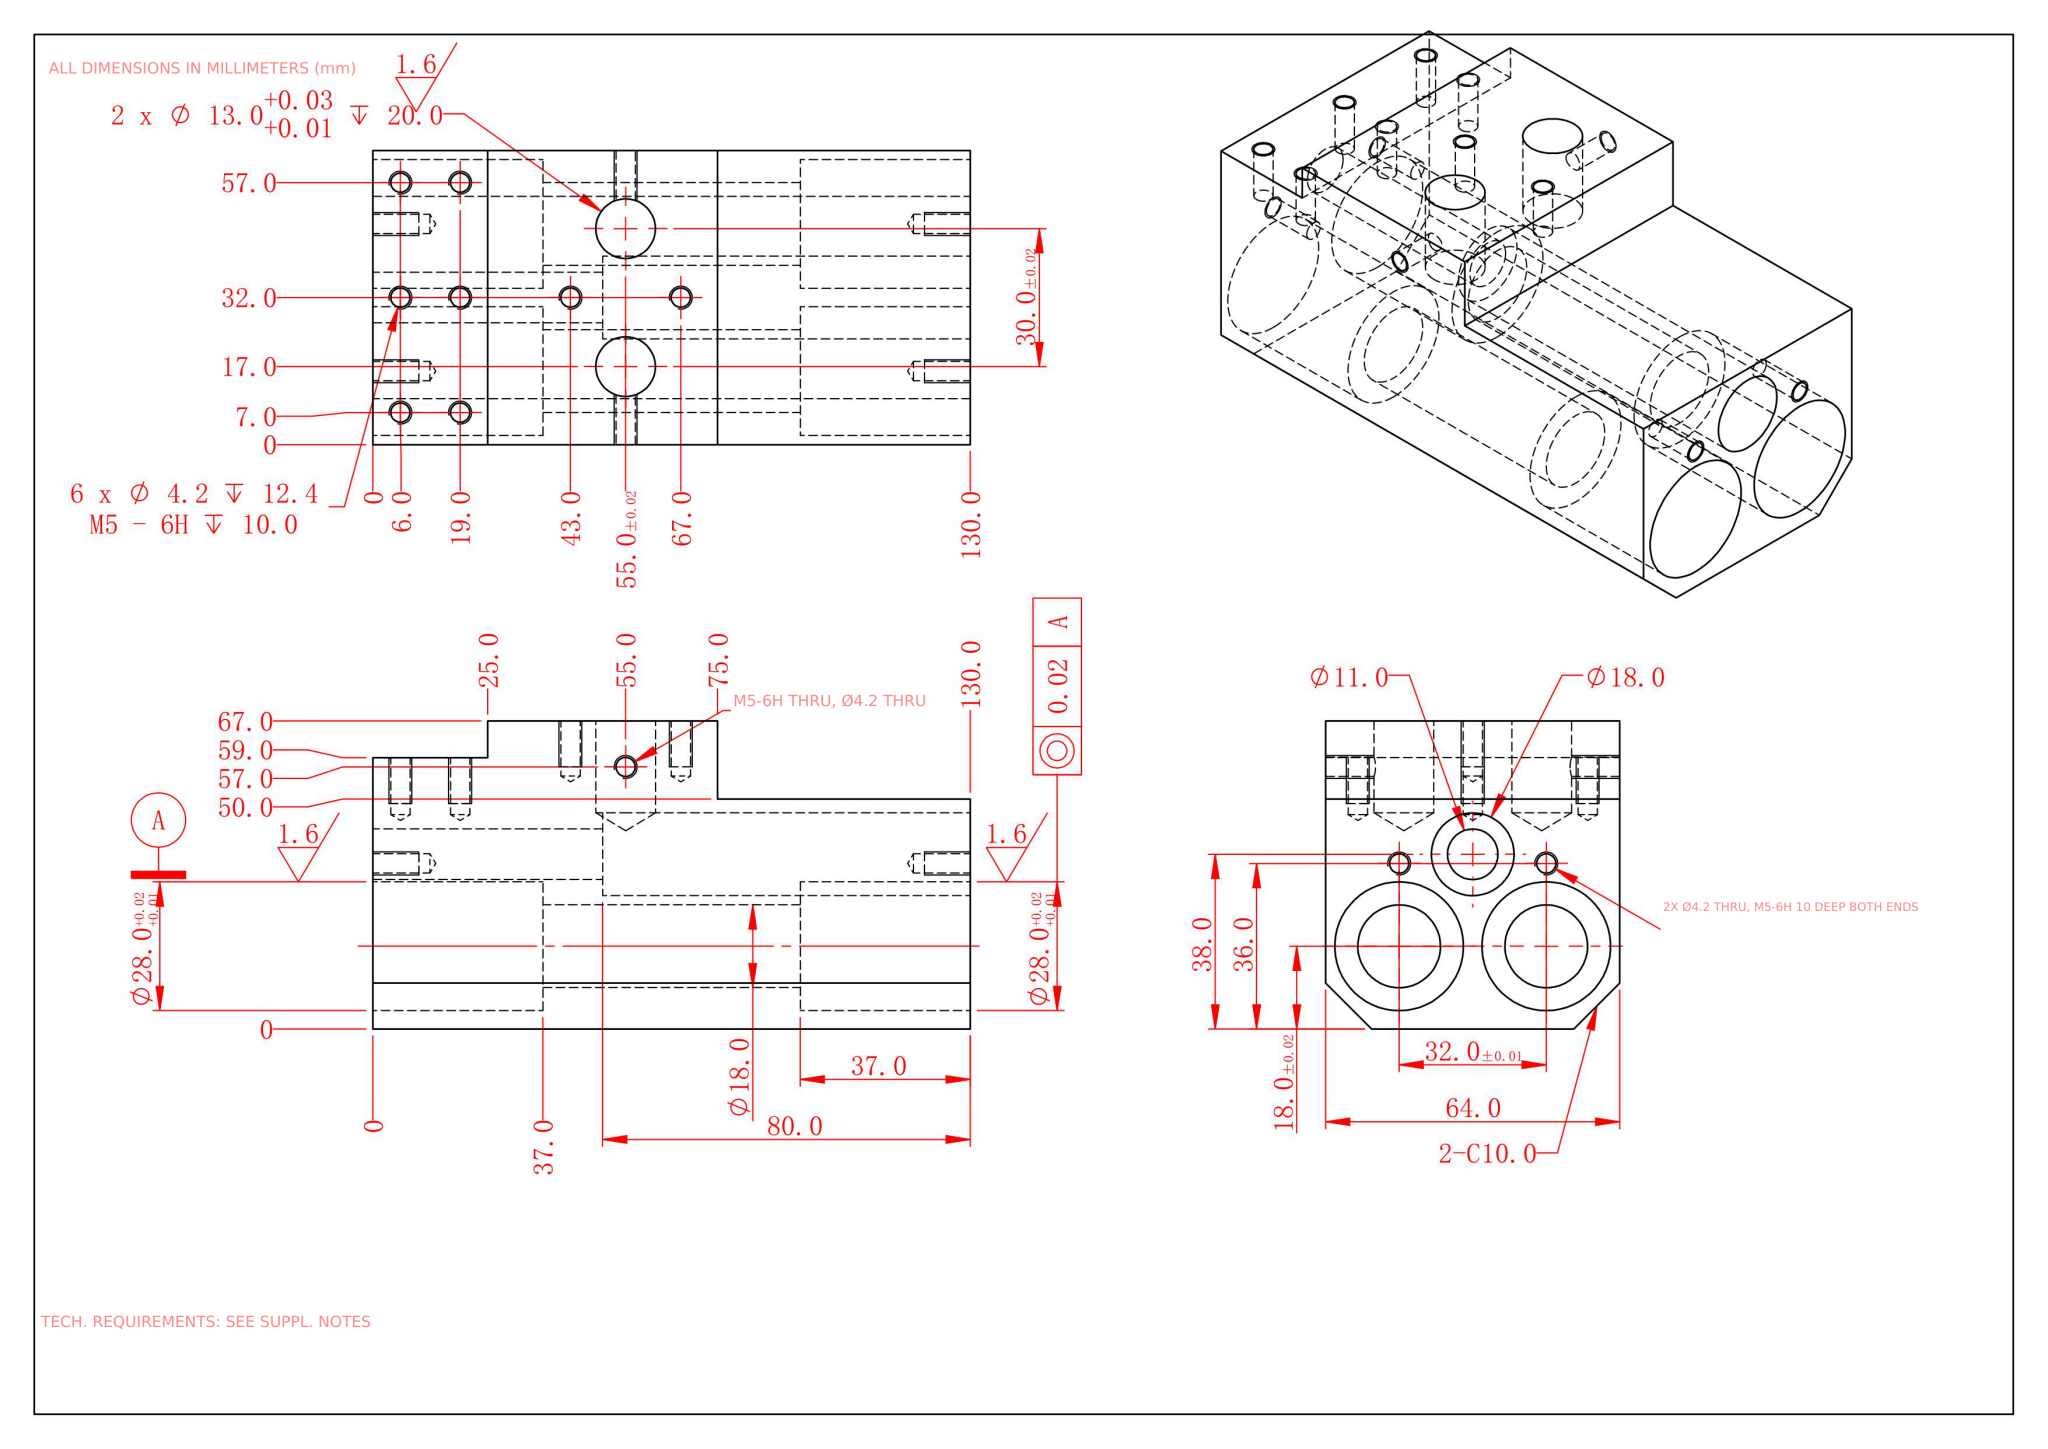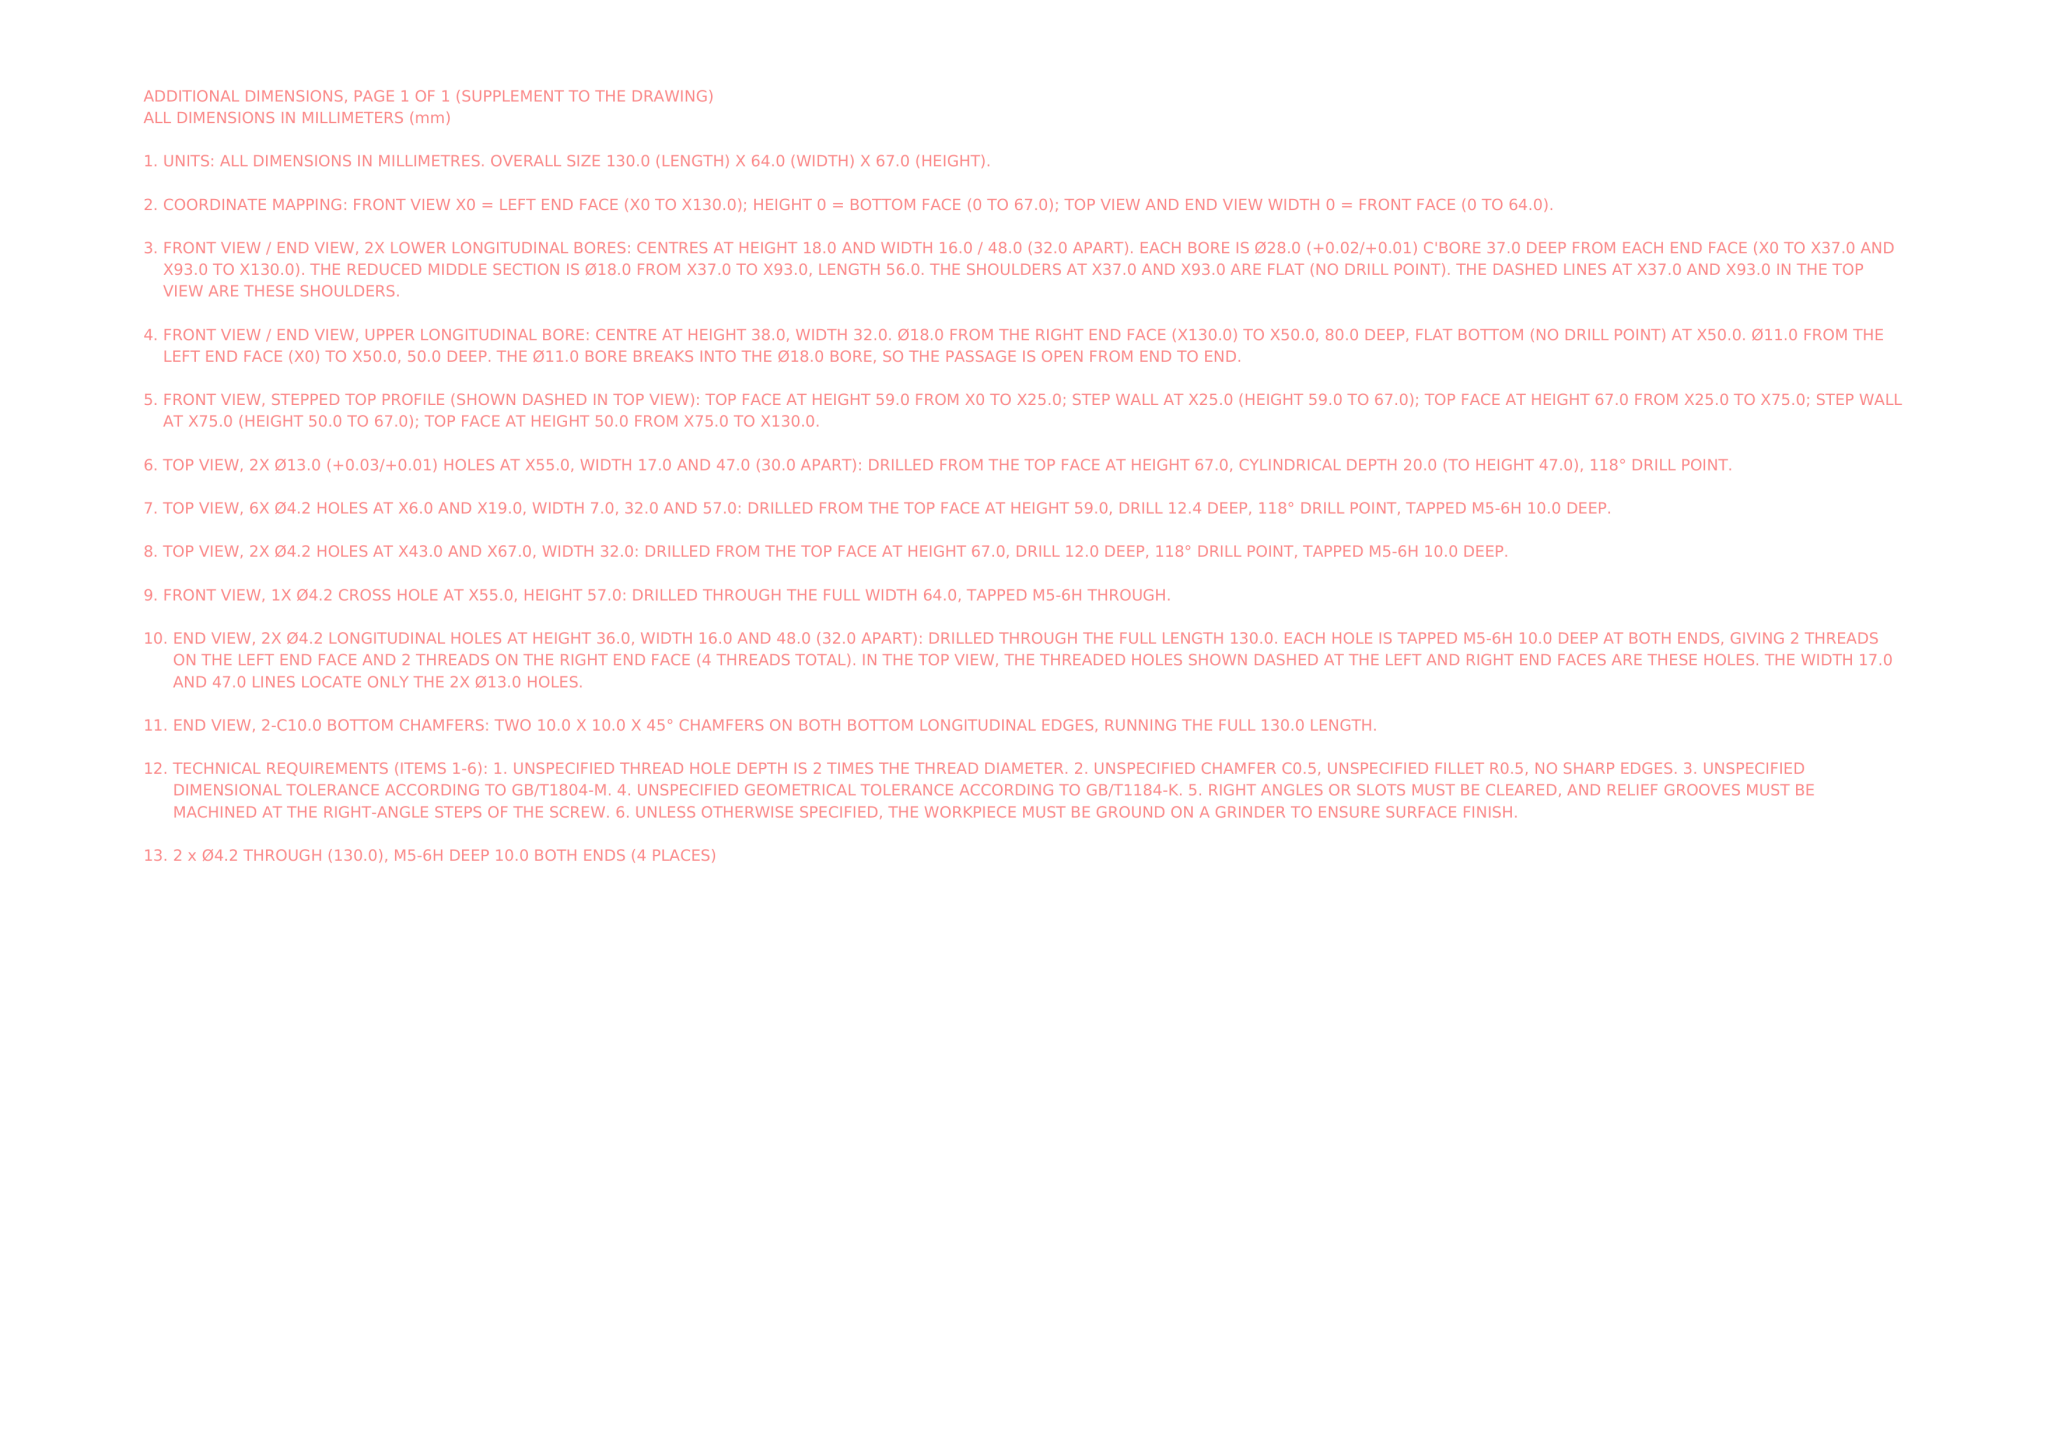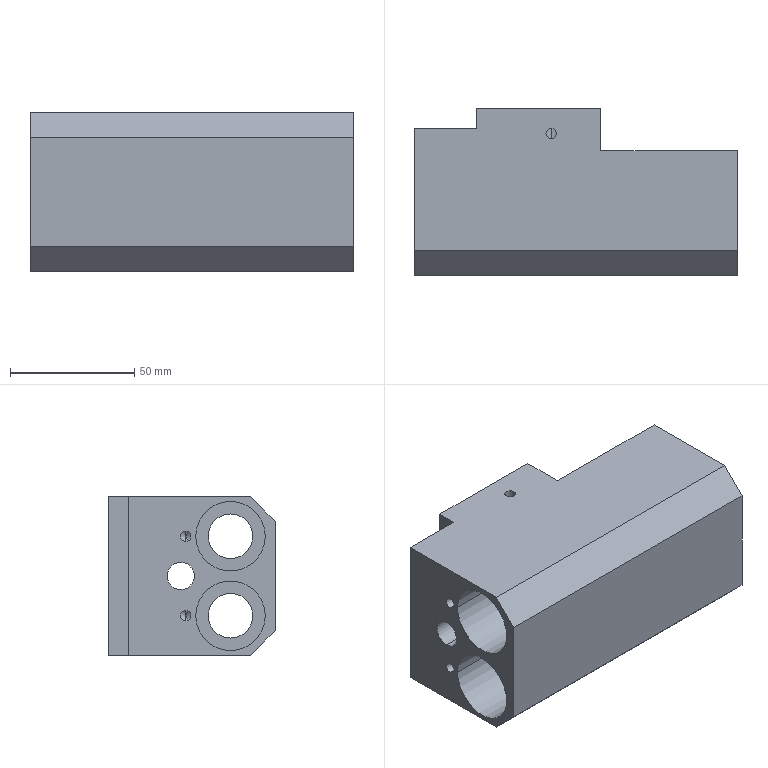Part | NX | mm | 1 solid | 93 faces | box 130 x 67 x 64 mm | volume 318990 mm3 | cylinder 48 | cone 28 | plane 17 | commonest cylinder face diameters 4.2 x28 28 x8 18 x6 13 x4 11 x2